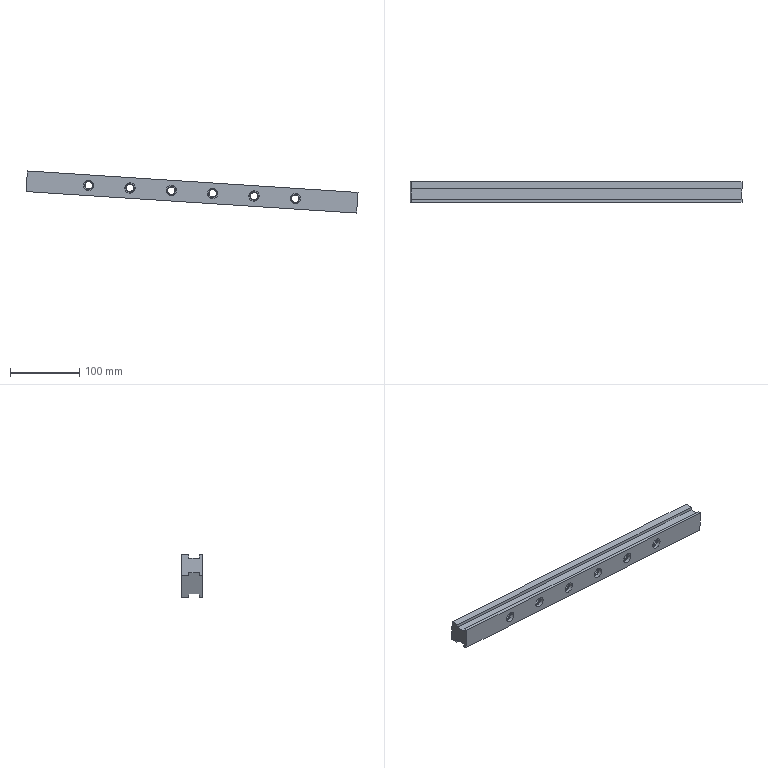Component | SolidWorks | GuideRail2-2 | 1 solid | 56 faces | box 480.94 x 30 x 61.01 mm | volume 349554 mm3 | cylinder 24 | plane 20 | cone 12 | commonest cylinder face diameters 10.2 x12 15 x12
build123d program:
from build123d import *

# Parameters (mm, degrees)
SKETCH1_W                    = 360
SKETCH1_H                    = 30
BOSS_EXTRUDE1_DEPTH          = 30
CUT_EXTRUDE1_DEPTH           = 585.893
CUT_EXTRUDE1_DEPTH_BACK      = 585.893
SKETCH2_W                    = 15
SKETCH2_H                    = 9
SKETCH3_R                    = 7.5
CUT_EXTRUDE2_DEPTH           = 5
M12_TAPPED_HOLE1_D           = 10.2
M12_TAPPED_HOLE1_DEPTH       = 50
M12_TAPPED_HOLE1_CSINK_D     = 12.05
M12_TAPPED_HOLE1_CSINK_ANGLE = 90
M12_TAPPED_HOLE1_TIP         = 3.064
BOSS_EXTRUDE2_DEPTH          = 60
BOSS_EXTRUDE3_START          = -360
BOSS_EXTRUDE3_DEPTH          = 60


with BuildPart() as part:
    # Sketch1 → Boss-Extrude1 (new body)
    with BuildSketch(Plane.XY):
        with Locations((-3.755, 445)):
            Rectangle(SKETCH1_W, SKETCH1_H)
    extrude(amount=BOSS_EXTRUDE1_DEPTH)

    # Sketch2 → Cut-Extrude1 (cut, two sides: drawn at the far end of the back side and taken through both)
    with BuildSketch(Plane.ZY.offset(183.755).offset(-CUT_EXTRUDE1_DEPTH_BACK)):
        with Locations((18, 460)):
            Rectangle(SKETCH2_W, SKETCH2_H)
        with Locations((18, 430)):
            Rectangle(SKETCH2_W, SKETCH2_H)
    extrude(amount=CUT_EXTRUDE1_DEPTH + CUT_EXTRUDE1_DEPTH_BACK, mode=Mode.SUBTRACT)

    # Sketch3 → Cut-Extrude2 (cut)
    with BuildSketch(Plane.XY.offset(30)):
        with Locations((146.245, 445)):
            Circle(SKETCH3_R)
        with Locations((86.245, 445)):
            Circle(SKETCH3_R)
        with Locations((26.245, 445)):
            Circle(SKETCH3_R)
        with Locations((-33.755, 445)):
            Circle(SKETCH3_R)
        with Locations((-93.755, 445)):
            Circle(SKETCH3_R)
        with Locations((-153.755, 445)):
            Circle(SKETCH3_R)
    extrude(amount=-CUT_EXTRUDE2_DEPTH, mode=Mode.SUBTRACT)

    # M12 Tapped Hole1
    with Locations(Plane(origin=(146.245, 445, 25), x_dir=(1, 0, 0), z_dir=(0, 0, 1))):
        with Locations((0, 0), (-60, 0), (-120, 0), (-180, 0), (-240, 0), (-300, 0)):
            CounterSinkHole(M12_TAPPED_HOLE1_D / 2, M12_TAPPED_HOLE1_CSINK_D / 2, depth=M12_TAPPED_HOLE1_DEPTH, counter_sink_angle=M12_TAPPED_HOLE1_CSINK_ANGLE)
            with Locations((0, 0, -(M12_TAPPED_HOLE1_DEPTH + M12_TAPPED_HOLE1_TIP / 2))):  # 118° drill point
                Cone(0, M12_TAPPED_HOLE1_D / 2, M12_TAPPED_HOLE1_TIP, mode=Mode.SUBTRACT)

    # Sketch5_2 → Boss-Extrude2 (add)
    with BuildSketch(Plane(origin=(176.245, 0, 0), x_dir=(0, 0, -1), z_dir=(1, 0, 0))):
        Polygon((0, 460), (-10.5, 460), (-10.5, 455.5), (-25.5, 455.5), (-25.5, 460), (-30, 460), (-30, 430), (-25.5, 430), (-25.5, 434.5), (-10.5, 434.5), (-10.5, 430), (0, 430), align=None)
    extrude(amount=BOSS_EXTRUDE2_DEPTH)

    # Sketch5_2 2 → Boss-Extrude3 (add)
    with BuildSketch(Plane(origin=(176.245, 0, 0), x_dir=(0, 0, -1), z_dir=(1, 0, 0)).offset(BOSS_EXTRUDE3_START)):
        Polygon((0, 460), (-10.5, 460), (-10.5, 455.5), (-25.5, 455.5), (-25.5, 460), (-30, 460), (-30, 430), (-25.5, 430), (-25.5, 434.5), (-10.5, 434.5), (-10.5, 430), (0, 430), align=None)
    extrude(amount=-BOSS_EXTRUDE3_DEPTH)


solid = part.part

# Placed as in the assembly
solid = solid.moved(Location((-17.932, -696, -634.403), (90, 0, -3.712)))